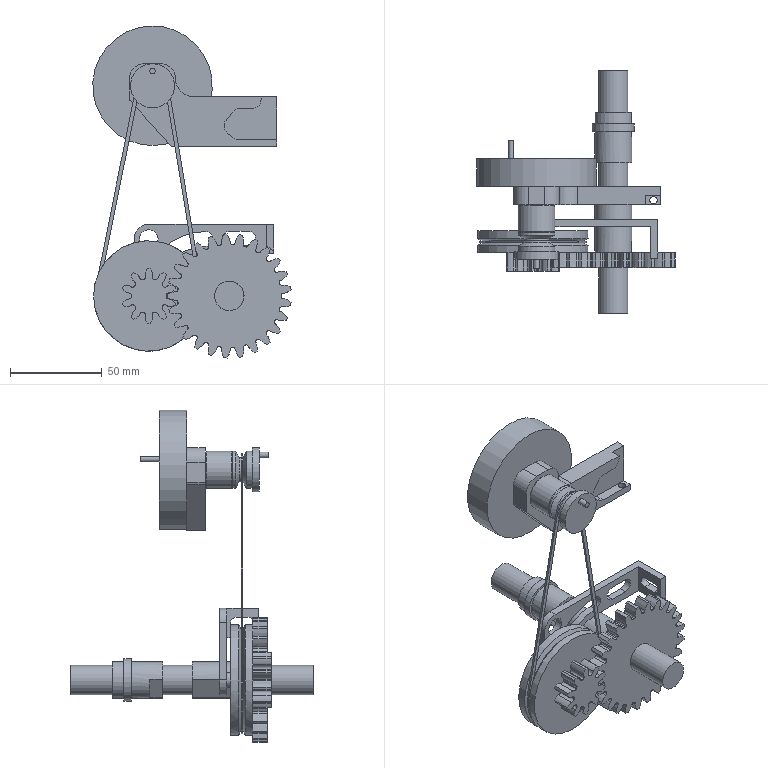Assembly | NX | mm | 8 component files | 11 solids | 363 faces | box 107.84 x 132 x 180.49 mm | volume 176325 mm3 | other 125 | cylinder 97 | plane 74 | spline 60 | cone 7 | commonest cylinder face diameters 56.25 x25 10 x15 18.71 x10 16 x8 20 x7 8 x6 8.5 x4 4 x2
Bill of materials:
unnamed part 1 | 1 |  | Thin closed loop band shaped like a teardrop: a large rounded end, a smaller rounded end, and two nearly straight tapering sides.
unnamed part 2 | 1 |  | Turned stud with a central cylindrical collar and a threaded shank on each end. The two shanks have different lengths, and each has a plain unthreaded neck next to the collar.
unnamed part 3 | 1 |  | Pulley-like body that turns about one axis. It has a V-shaped circumferential groove between two flanges, a larger stepped base flange, and a small cylindrical pin standing off the flat outer face.
unnamed part 4 | 1 |  | Flat circular disc with a small threaded-looking hole on one face and a small slender cylindrical pin protruding from the other face, offset from the centre.
unnamed part 5 | 1 |  | Bent flat-plate L-shaped bracket. The main plate has a round hole, a long curved arc slot and a straight slot, and a short flange is bent at 90 degrees with its own straight slot.
unnamed part 6 | 1 |  | Thick plate lever or arm. A rounded raised lug at one end has a through-hole, a long flat body has an angled chamfered edge, and a curved cutout or step at the far end has a small cross-hole.
unnamed part 7 | 1 |  | Combined body: a spur-type gear with about 25 teeth and a central bore, overlapping and offset from a larger disc or wheel that has a circumferential groove and a small hub. A second toothed feature appears to sit behind or within the large disc.
unnamed part 8 | 1 |  | Solid stepped round shaft with several diameter sections along its length, including two larger raised bands and a narrow ring or collar.
Mates:
1. fix | model3 1 component
2. touch align | model2 1 face | model1 1 face
3. touch align | model4 1 face | model1 1 face
4. touch align | model1 1 face | model4 1 face
5. touch align | model3 1 face | model2 1 face
6. touch align | model3 1 face | model2 1 face
7. touch align | model9 1 edge | model3 1 edge
8. touch align | model9 1 face | model3 1 edge
9. touch align | model6 1 edge | model9 1 edge
10. touch align | model9 1 face | model6 1 edge
11. touch align | model7 1 face | model6 1 edge
12. touch align | model6 1 face | model7 1 face
13. touch align | model5 1 face | model6 1 face
14. touch align | model6 1 face | model5 1 face
15. touch align | model2 1 face | model4 1 face